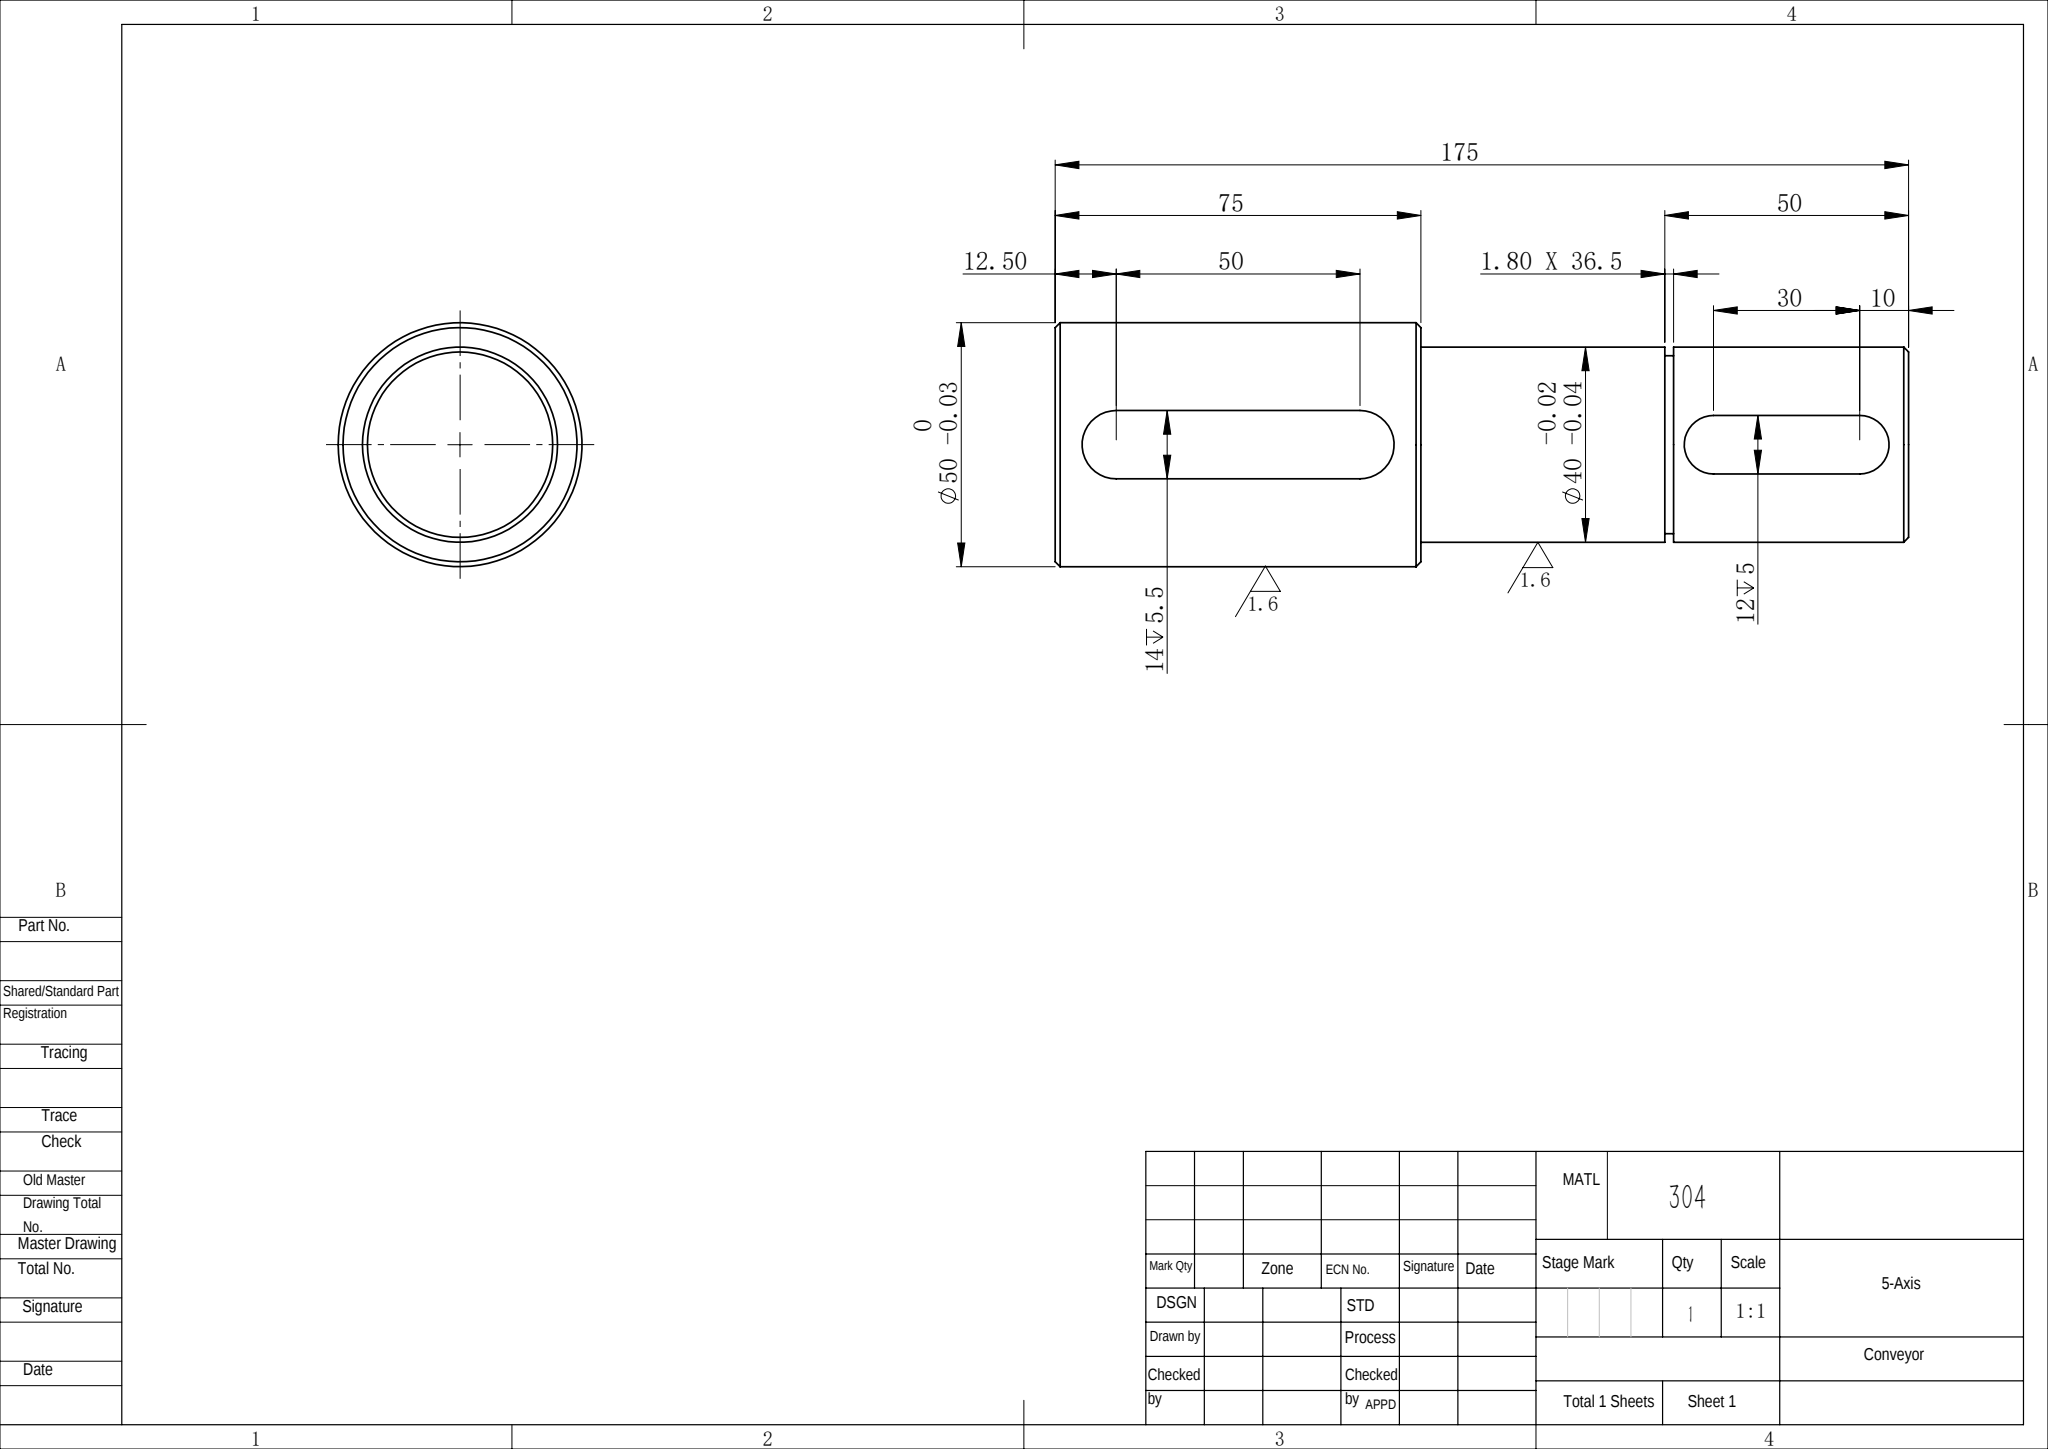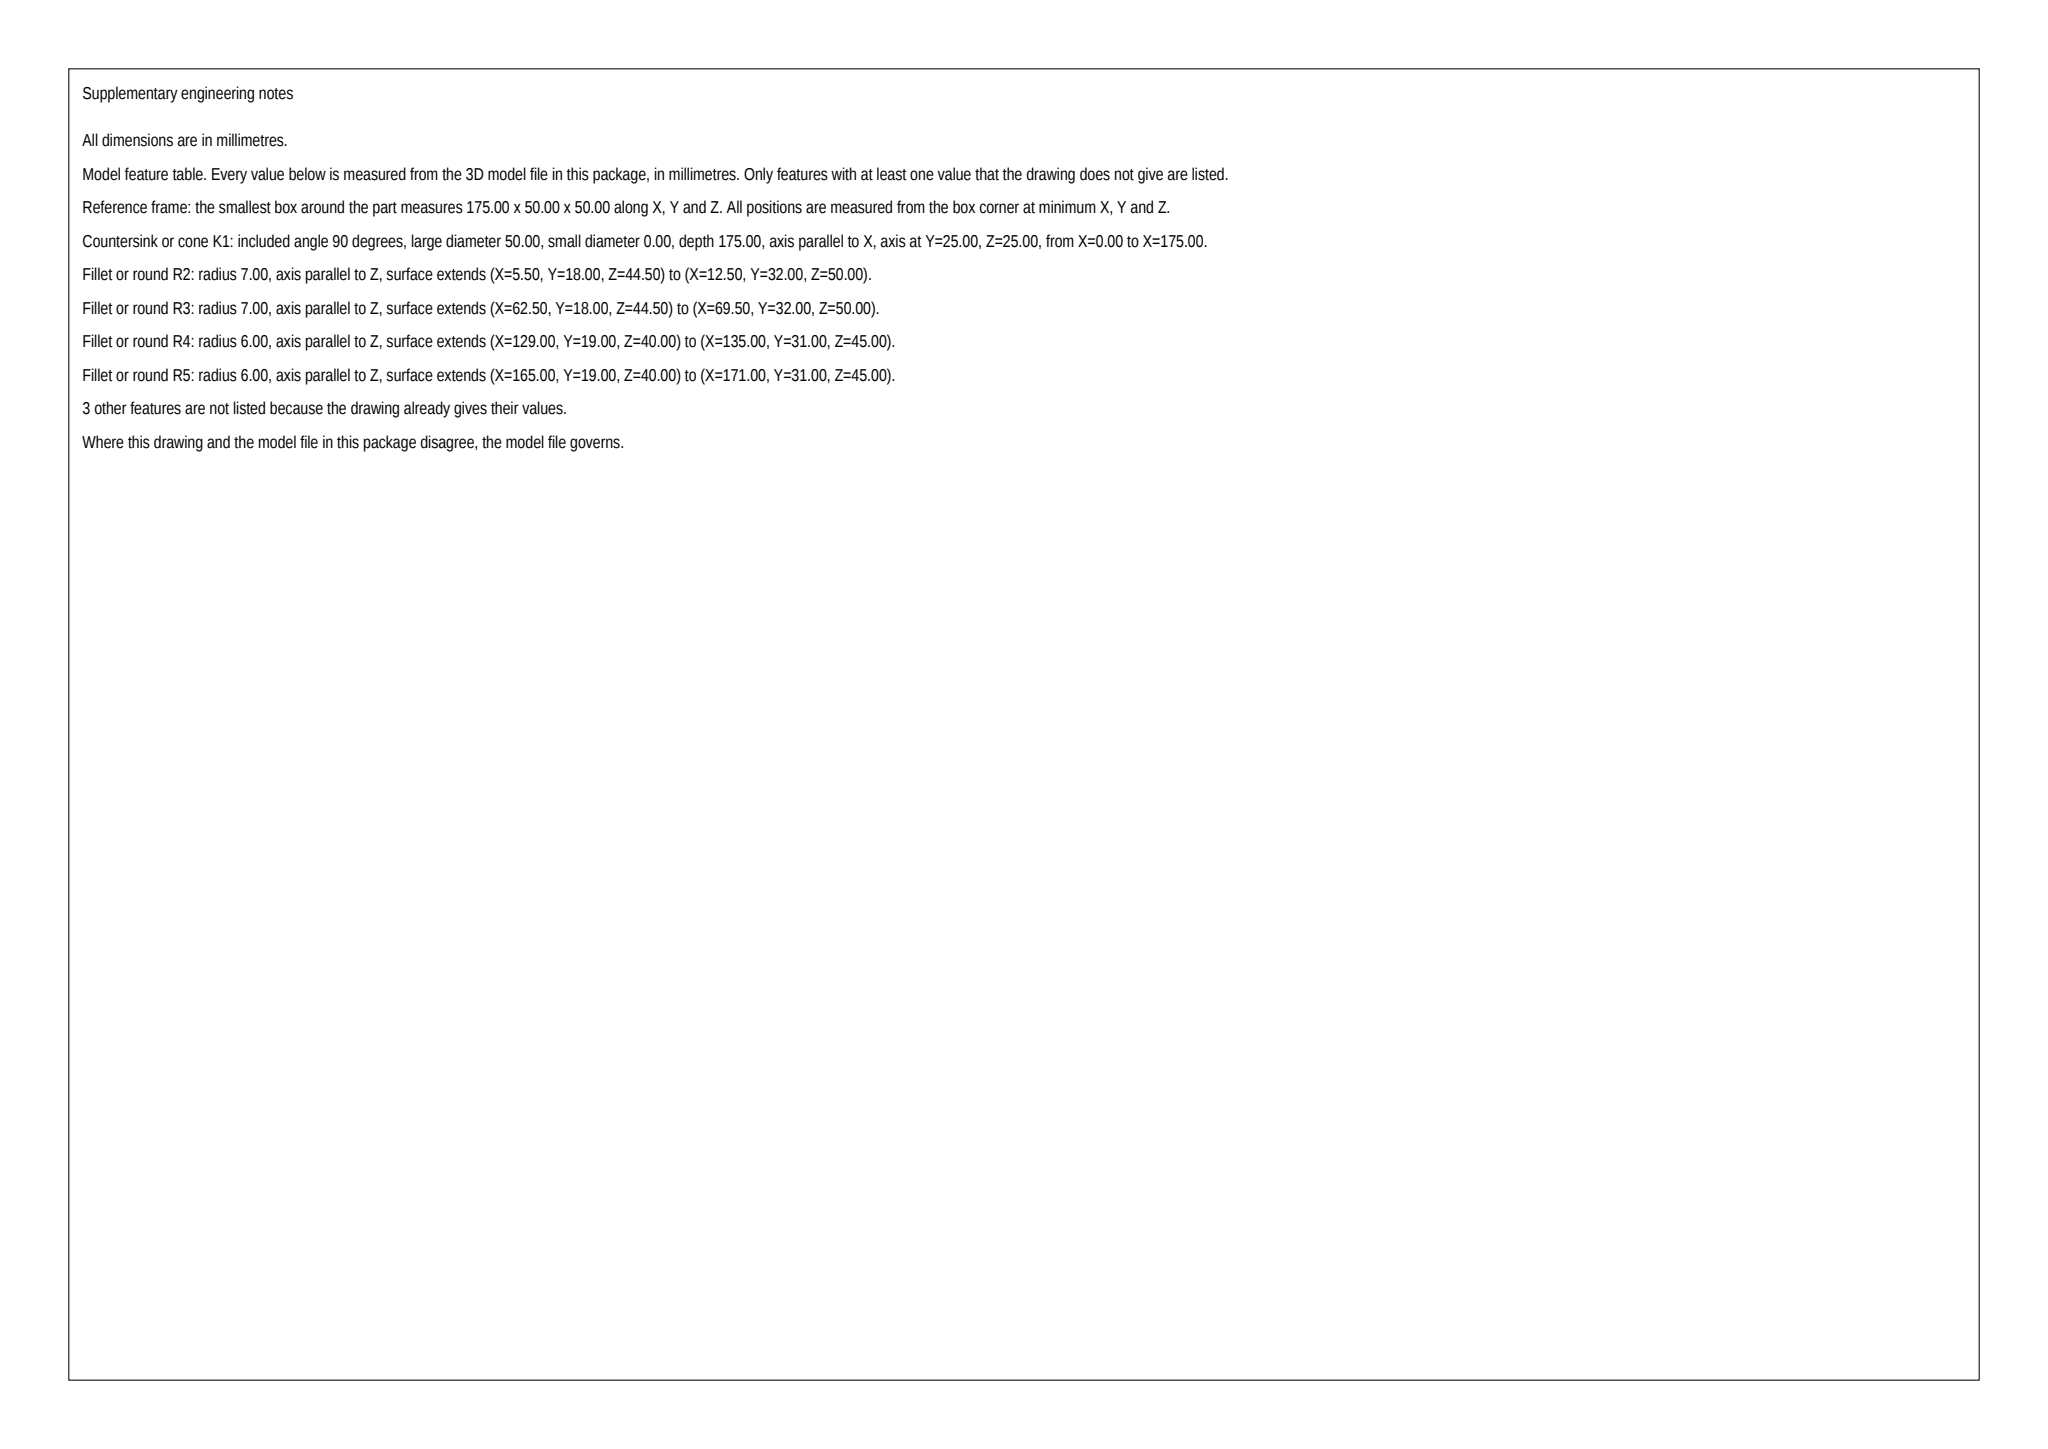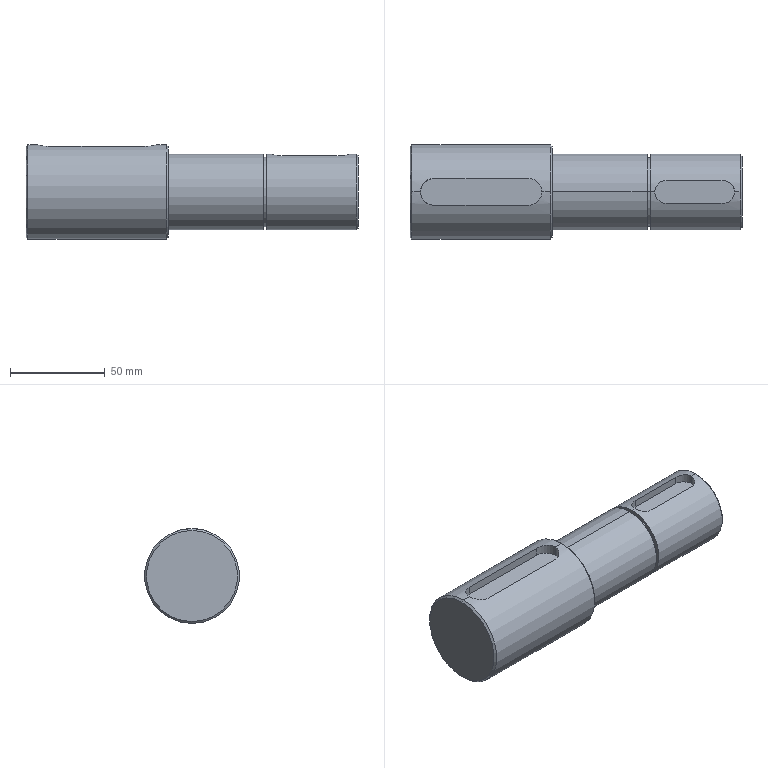Part | SolidWorks | mm | material 304 | 1 solid | 31 faces | box 175 x 50 x 50 mm | volume 265673 mm3 | cylinder 14 | plane 11 | cone 6 | commonest cylinder face diameters 40 x4 12 x3 14 x3 36.5 x2 50 x2
build123d program:
from build123d import *

# Parameters (mm, degrees)
CHAMFER1_SIZE      = 1
CUT_EXTRUDE1_DEPTH = 5
CUT_EXTRUDE2_DEPTH = 5.5
SKETCH4_W          = 1.8
SKETCH4_H          = 19.851


with BuildPart() as part:
    # Sketch1 → Revolve1 (revolve)
    with BuildSketch(Plane(origin=(0, 0, 0), x_dir=(1, 0, 0), z_dir=(0, 1, 0)), mode=Mode.PRIVATE) as revolve1_sk:
        Polygon((0, 0), (175, 0), (175, 20), (75, 20), (75, 25), (0, 25), align=None)
    revolve(revolve1_sk.sketch.rotate(Axis((0, 0, 0), (1, 0, 0)), 180), axis=Axis((0, 0, 0), (1, 0, 0)))

    # Chamfer1
    chamfer1_edges = [part.edges().sort_by_distance(p)[0] for p in [
        (0, 0, -25),
        (75, 0, -25),
        (175, 0, -20),
    ]]
    chamfer(chamfer1_edges, length=CHAMFER1_SIZE)

    # Sketch2 → Cut-Extrude1 (cut)
    with BuildSketch(Plane.XY.offset(20)):
        with BuildLine():
            Line((135, 6), (165, 6))
            ThreePointArc((165, 6), (171, 0), (165, -6))
            Line((165, -6), (135, -6))
            ThreePointArc((135, -6), (129, 0), (135, 6))
        make_face()
    extrude(amount=-CUT_EXTRUDE1_DEPTH, mode=Mode.SUBTRACT)

    # Sketch3 → Cut-Extrude2 (cut)
    with BuildSketch(Plane.XY.offset(25)):
        with BuildLine():
            Line((12.5, 7), (62.5, 7))
            ThreePointArc((62.5, 7), (69.5, 0), (62.5, -7))
            Line((62.5, -7), (12.5, -7))
            ThreePointArc((12.5, -7), (5.5, 0), (12.5, 7))
        make_face()
    extrude(amount=-CUT_EXTRUDE2_DEPTH, mode=Mode.SUBTRACT)

    # Sketch4 → Cut-Revolve1 (revolve, cut)
    with BuildSketch(Plane.XY, mode=Mode.PRIVATE) as cut_revolve1_sk:
        with Locations((125.9, 28.176)):
            Rectangle(SKETCH4_W, SKETCH4_H)
    revolve(cut_revolve1_sk.sketch.rotate(Axis((0, 0, 0), (1, 0, 0)), 90), axis=Axis((0, 0, 0), (1, 0, 0)), mode=Mode.SUBTRACT)


solid = part.part